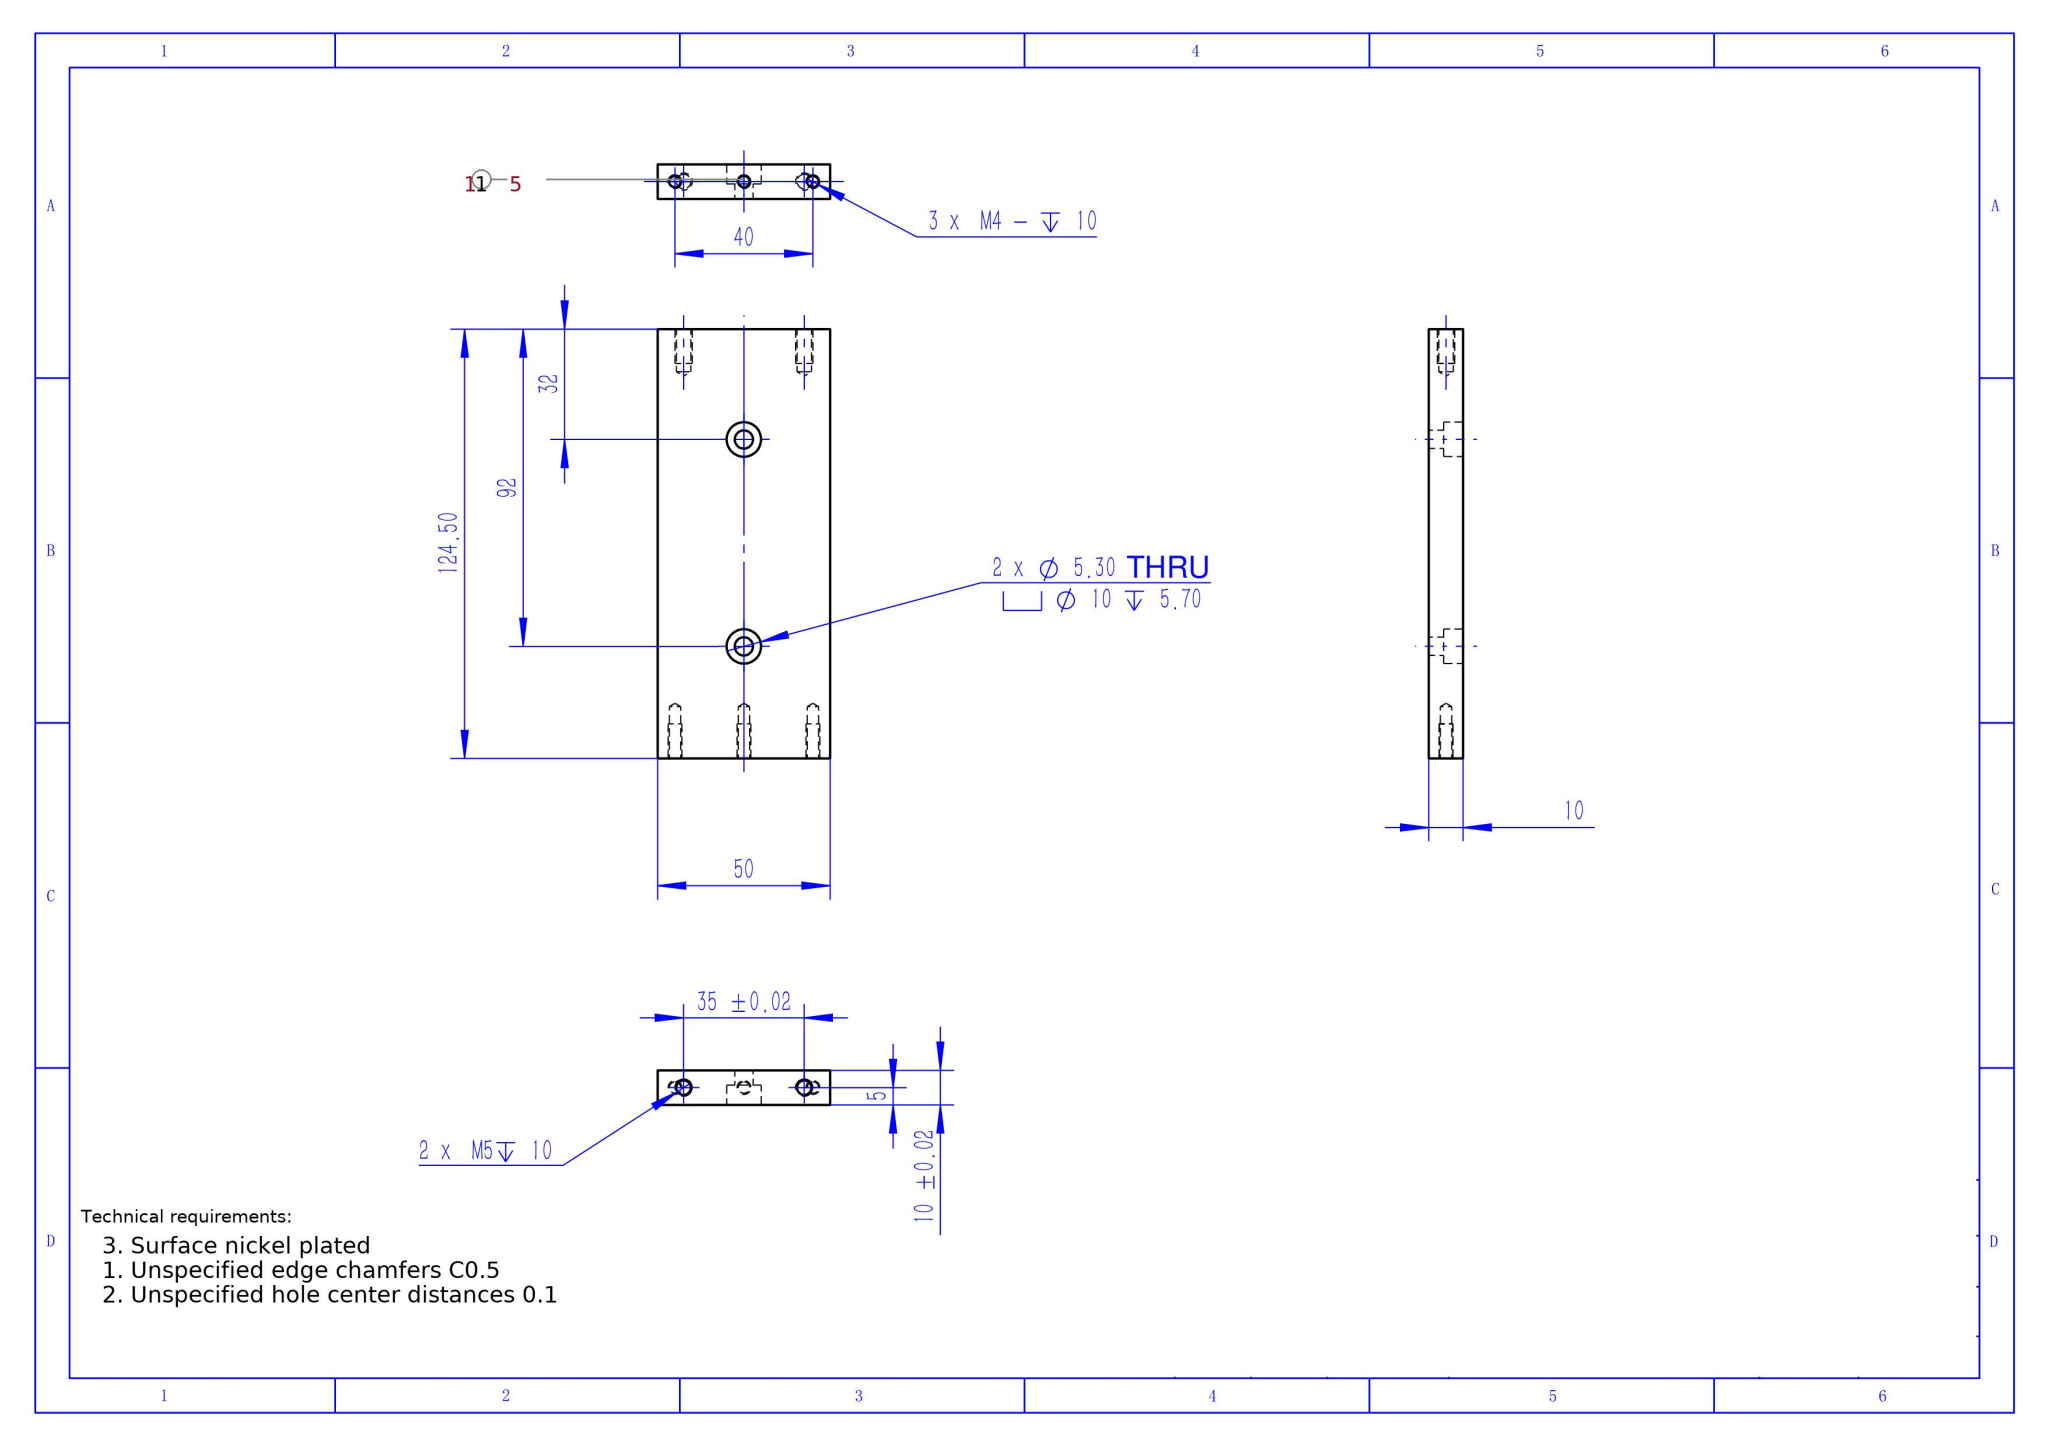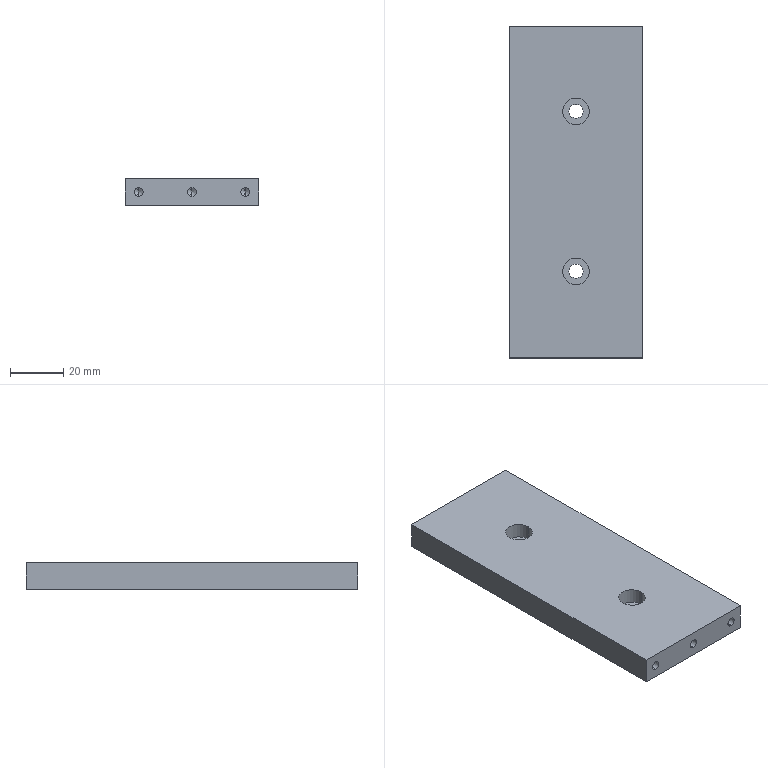Part | SolidWorks | mm | 1 solid | 36 faces | box 50 x 124.5 x 10 mm | volume 60416 mm3 | cylinder 18 | cone 10 | plane 8 | commonest cylinder face diameters 3.3 x6 10 x4 5.3 x4 4.2 x4
build123d program:
from build123d import *

# Parameters (mm, degrees)
SKETCH1_W                                         = 50
SKETCH1_H                                         = 124.5
BOSS_EXTRUDE1_DEPTH                               = 10
M5_TAPPED_HOLE1_D                                 = 4.2
M5_TAPPED_HOLE1_DEPTH                             = 12.4
M5_TAPPED_HOLE1_TIP                               = 1.262
HOLE_SIZE_ACCORDING_TO_HEX_SOCKET_HEA_D           = 5.3
HOLE_SIZE_ACCORDING_TO_HEX_SOCKET_HEA_CBORE_D     = 10
HOLE_SIZE_ACCORDING_TO_HEX_SOCKET_HEA_CBORE_DEPTH = 5.7
M4_TAPPED_HOLE1_D                                 = 3.3
M4_TAPPED_HOLE1_DEPTH                             = 15
M4_TAPPED_HOLE1_TIP                               = 0.9914


with BuildPart() as part:
    # Sketch1 → Boss-Extrude1 (new body)
    with BuildSketch(Plane.XY):
        with Locations((0, -62.25)):
            Rectangle(SKETCH1_W, SKETCH1_H)
    extrude(amount=BOSS_EXTRUDE1_DEPTH)

    # M5 Tapped Hole1
    with Locations(Plane(origin=(0, 0, 0), x_dir=(1, 0, 0), z_dir=(0, 1, 0))):
        with Locations((17.5, -5), (-17.5, -5)):
            Hole(M5_TAPPED_HOLE1_D / 2, depth=M5_TAPPED_HOLE1_DEPTH)
            with Locations((0, 0, -(M5_TAPPED_HOLE1_DEPTH + M5_TAPPED_HOLE1_TIP / 2))):  # 118° drill point
                Cone(0, M5_TAPPED_HOLE1_D / 2, M5_TAPPED_HOLE1_TIP, mode=Mode.SUBTRACT)

    # Hole Size _ according to_ Hex Socket Hea (through all)
    with Locations(Plane(origin=(0, 0, 10), x_dir=(-1, 0, 0), z_dir=(0, 0, 1))):
        with Locations((0, 32), (0, 92)):
            CounterBoreHole(HOLE_SIZE_ACCORDING_TO_HEX_SOCKET_HEA_D / 2, HOLE_SIZE_ACCORDING_TO_HEX_SOCKET_HEA_CBORE_D / 2, HOLE_SIZE_ACCORDING_TO_HEX_SOCKET_HEA_CBORE_DEPTH)

    # M4 Tapped Hole1
    with Locations(Plane(origin=(20, -124.5, 5), x_dir=(0, 0, -1), z_dir=(0, -1, 0))):
        with Locations((0, 0), (0, -20), (0, -40)):
            Hole(M4_TAPPED_HOLE1_D / 2, depth=M4_TAPPED_HOLE1_DEPTH)
            with Locations((0, 0, -(M4_TAPPED_HOLE1_DEPTH + M4_TAPPED_HOLE1_TIP / 2))):  # 118° drill point
                Cone(0, M4_TAPPED_HOLE1_D / 2, M4_TAPPED_HOLE1_TIP, mode=Mode.SUBTRACT)


solid = part.part
STEP:
#1=CARTESIAN_POINT('',(20.,-109.5,6.65));
#2=VERTEX_POINT('',#1);
#3=CARTESIAN_POINT('',(20.,-109.5,3.35));
#4=VERTEX_POINT('',#3);
#5=CARTESIAN_POINT('',(20.,-109.5,5.));
#6=DIRECTION('',(0.,-1.,0.));
#7=DIRECTION('',(0.,0.,-1.));
#8=AXIS2_PLACEMENT_3D('',#5,#6,#7);
#9=CIRCLE('',#8,1.65);
#10=EDGE_CURVE('',#2,#4,#9,.T.);
#11=ORIENTED_EDGE('',*,*,#10,.F.);
#12=CARTESIAN_POINT('',(20.,-124.5,6.65));
#13=VERTEX_POINT('',#12);
#14=CARTESIAN_POINT('',(20.,-124.5,6.65));
#15=DIRECTION('',(0.,-1.,0.));
#16=VECTOR('',#15,1000.);
#17=LINE('',#14,#16);
#18=EDGE_CURVE('',#2,#13,#17,.T.);
#19=ORIENTED_EDGE('',*,*,#18,.T.);
#20=CARTESIAN_POINT('',(20.,-124.5,3.35));
#21=VERTEX_POINT('',#20);
#22=CARTESIAN_POINT('',(20.,-124.5,5.));
#23=DIRECTION('',(0.,-1.,0.));
#24=DIRECTION('',(0.,0.,-1.));
#25=AXIS2_PLACEMENT_3D('',#22,#23,#24);
#26=CIRCLE('',#25,1.65);
#27=EDGE_CURVE('',#13,#21,#26,.T.);
#28=ORIENTED_EDGE('',*,*,#27,.T.);
#29=CARTESIAN_POINT('',(20.,-124.5,3.35));
#30=DIRECTION('',(0.,-1.,0.));
#31=VECTOR('',#30,1000.);
#32=LINE('',#29,#31);
#33=EDGE_CURVE('',#4,#21,#32,.T.);
#34=ORIENTED_EDGE('',*,*,#33,.F.);
#35=EDGE_LOOP('',(#11,#19,#28,#34));
#36=FACE_OUTER_BOUND('',#35,.T.);
#37=CARTESIAN_POINT('',(20.,-124.5,5.));
#38=DIRECTION('',(0.,-1.,0.));
#39=DIRECTION('',(0.,0.,-1.));
#40=AXIS2_PLACEMENT_3D('',#37,#38,#39);
#41=CYLINDRICAL_SURFACE('',#40,1.65);
#42=ADVANCED_FACE('',(#36),#41,.F.);
#43=CARTESIAN_POINT('',(20.,-108.509,5.));
#44=VERTEX_POINT('',#43);
#45=CARTESIAN_POINT('',(20.,-109.5,3.35));
#46=DIRECTION('',(0.,-0.515,-0.8572));
#47=VECTOR('',#46,1000.);
#48=LINE('',#45,#47);
#49=EDGE_CURVE('',#44,#4,#48,.T.);
#50=ORIENTED_EDGE('',*,*,#49,.F.);
#51=CARTESIAN_POINT('',(20.,-109.5,6.65));
#52=DIRECTION('',(0.,-0.515,0.8572));
#53=VECTOR('',#52,1000.);
#54=LINE('',#51,#53);
#55=EDGE_CURVE('',#44,#2,#54,.T.);
#56=ORIENTED_EDGE('',*,*,#55,.T.);
#57=ORIENTED_EDGE('',*,*,#10,.T.);
#58=EDGE_LOOP('',(#50,#56,#57));
#59=FACE_OUTER_BOUND('',#58,.T.);
#60=CARTESIAN_POINT('',(20.,-109.5,5.));
#61=DIRECTION('',(0.,-1.,0.));
#62=DIRECTION('',(0.,0.,-1.));
#63=AXIS2_PLACEMENT_3D('',#60,#61,#62);
#64=CONICAL_SURFACE('',#63,1.65,1.03);
#65=ADVANCED_FACE('',(#59),#64,.F.);
#66=CARTESIAN_POINT('',(-0.,-109.5,6.65));
#67=VERTEX_POINT('',#66);
#68=CARTESIAN_POINT('',(-0.,-109.5,3.35));
#69=VERTEX_POINT('',#68);
#70=CARTESIAN_POINT('',(-0.,-109.5,5.));
#71=DIRECTION('',(0.,-1.,0.));
#72=DIRECTION('',(0.,0.,-1.));
#73=AXIS2_PLACEMENT_3D('',#70,#71,#72);
#74=CIRCLE('',#73,1.65);
#75=EDGE_CURVE('',#67,#69,#74,.T.);
#76=ORIENTED_EDGE('',*,*,#75,.F.);
#77=CARTESIAN_POINT('',(-0.,-124.5,6.65));
#78=VERTEX_POINT('',#77);
#79=CARTESIAN_POINT('',(-0.,-124.5,6.65));
#80=DIRECTION('',(0.,-1.,0.));
#81=VECTOR('',#80,1000.);
#82=LINE('',#79,#81);
#83=EDGE_CURVE('',#67,#78,#82,.T.);
#84=ORIENTED_EDGE('',*,*,#83,.T.);
#85=CARTESIAN_POINT('',(-0.,-124.5,3.35));
#86=VERTEX_POINT('',#85);
#87=CARTESIAN_POINT('',(-0.,-124.5,5.));
#88=DIRECTION('',(0.,-1.,0.));
#89=DIRECTION('',(0.,0.,-1.));
#90=AXIS2_PLACEMENT_3D('',#87,#88,#89);
#91=CIRCLE('',#90,1.65);
#92=EDGE_CURVE('',#78,#86,#91,.T.);
#93=ORIENTED_EDGE('',*,*,#92,.T.);
#94=CARTESIAN_POINT('',(-0.,-124.5,3.35));
#95=DIRECTION('',(0.,-1.,0.));
#96=VECTOR('',#95,1000.);
#97=LINE('',#94,#96);
#98=EDGE_CURVE('',#69,#86,#97,.T.);
#99=ORIENTED_EDGE('',*,*,#98,.F.);
#100=EDGE_LOOP('',(#76,#84,#93,#99));
#101=FACE_OUTER_BOUND('',#100,.T.);
#102=CARTESIAN_POINT('',(-0.,-124.5,5.));
#103=DIRECTION('',(0.,-1.,0.));
#104=DIRECTION('',(0.,0.,-1.));
#105=AXIS2_PLACEMENT_3D('',#102,#103,#104);
#106=CYLINDRICAL_SURFACE('',#105,1.65);
#107=ADVANCED_FACE('',(#101),#106,.F.);
#108=CARTESIAN_POINT('',(-0.,-108.509,5.));
#109=VERTEX_POINT('',#108);
#110=CARTESIAN_POINT('',(-0.,-109.5,3.35));
#111=DIRECTION('',(0.,-0.515,-0.8572));
#112=VECTOR('',#111,1000.);
#113=LINE('',#110,#112);
#114=EDGE_CURVE('',#109,#69,#113,.T.);
#115=ORIENTED_EDGE('',*,*,#114,.F.);
#116=CARTESIAN_POINT('',(-0.,-109.5,6.65));
#117=DIRECTION('',(0.,-0.515,0.8572));
#118=VECTOR('',#117,1000.);
#119=LINE('',#116,#118);
#120=EDGE_CURVE('',#109,#67,#119,.T.);
#121=ORIENTED_EDGE('',*,*,#120,.T.);
#122=ORIENTED_EDGE('',*,*,#75,.T.);
#123=EDGE_LOOP('',(#115,#121,#122));
#124=FACE_OUTER_BOUND('',#123,.T.);
#125=CARTESIAN_POINT('',(-0.,-109.5,5.));
#126=DIRECTION('',(0.,-1.,0.));
#127=DIRECTION('',(0.,0.,-1.));
#128=AXIS2_PLACEMENT_3D('',#125,#126,#127);
#129=CONICAL_SURFACE('',#128,1.65,1.03);
#130=ADVANCED_FACE('',(#124),#129,.F.);
#131=CARTESIAN_POINT('',(-20.,-109.5,6.65));
#132=VERTEX_POINT('',#131);
#133=CARTESIAN_POINT('',(-20.,-109.5,3.35));
#134=VERTEX_POINT('',#133);
#135=CARTESIAN_POINT('',(-20.,-109.5,5.));
#136=DIRECTION('',(0.,-1.,0.));
#137=DIRECTION('',(0.,0.,-1.));
#138=AXIS2_PLACEMENT_3D('',#135,#136,#137);
#139=CIRCLE('',#138,1.65);
#140=EDGE_CURVE('',#132,#134,#139,.T.);
#141=ORIENTED_EDGE('',*,*,#140,.F.);
#142=CARTESIAN_POINT('',(-20.,-124.5,6.65));
#143=VERTEX_POINT('',#142);
#144=CARTESIAN_POINT('',(-20.,-124.5,6.65));
#145=DIRECTION('',(0.,-1.,0.));
#146=VECTOR('',#145,1000.);
#147=LINE('',#144,#146);
#148=EDGE_CURVE('',#132,#143,#147,.T.);
#149=ORIENTED_EDGE('',*,*,#148,.T.);
#150=CARTESIAN_POINT('',(-20.,-124.5,3.35));
#151=VERTEX_POINT('',#150);
#152=CARTESIAN_POINT('',(-20.,-124.5,5.));
#153=DIRECTION('',(0.,-1.,0.));
#154=DIRECTION('',(0.,0.,-1.));
#155=AXIS2_PLACEMENT_3D('',#152,#153,#154);
#156=CIRCLE('',#155,1.65);
#157=EDGE_CURVE('',#143,#151,#156,.T.);
#158=ORIENTED_EDGE('',*,*,#157,.T.);
#159=CARTESIAN_POINT('',(-20.,-124.5,3.35));
#160=DIRECTION('',(0.,-1.,0.));
#161=VECTOR('',#160,1000.);
#162=LINE('',#159,#161);
#163=EDGE_CURVE('',#134,#151,#162,.T.);
#164=ORIENTED_EDGE('',*,*,#163,.F.);
#165=EDGE_LOOP('',(#141,#149,#158,#164));
#166=FACE_OUTER_BOUND('',#165,.T.);
#167=CARTESIAN_POINT('',(-20.,-124.5,5.));
#168=DIRECTION('',(0.,-1.,0.));
#169=DIRECTION('',(0.,0.,-1.));
#170=AXIS2_PLACEMENT_3D('',#167,#168,#169);
#171=CYLINDRICAL_SURFACE('',#170,1.65);
#172=ADVANCED_FACE('',(#166),#171,.F.);
#173=CARTESIAN_POINT('',(-20.,-108.509,5.));
#174=VERTEX_POINT('',#173);
#175=CARTESIAN_POINT('',(-20.,-109.5,3.35));
#176=DIRECTION('',(0.,-0.515,-0.8572));
#177=VECTOR('',#176,1000.);
#178=LINE('',#175,#177);
#179=EDGE_CURVE('',#174,#134,#178,.T.);
#180=ORIENTED_EDGE('',*,*,#179,.F.);
#181=CARTESIAN_POINT('',(-20.,-109.5,6.65));
#182=DIRECTION('',(0.,-0.515,0.8572));
#183=VECTOR('',#182,1000.);
#184=LINE('',#181,#183);
#185=EDGE_CURVE('',#174,#132,#184,.T.);
#186=ORIENTED_EDGE('',*,*,#185,.T.);
#187=ORIENTED_EDGE('',*,*,#140,.T.);
#188=EDGE_LOOP('',(#180,#186,#187));
#189=FACE_OUTER_BOUND('',#188,.T.);
#190=CARTESIAN_POINT('',(-20.,-109.5,5.));
#191=DIRECTION('',(0.,-1.,0.));
#192=DIRECTION('',(0.,0.,-1.));
#193=AXIS2_PLACEMENT_3D('',#190,#191,#192);
#194=CONICAL_SURFACE('',#193,1.65,1.03);
#195=ADVANCED_FACE('',(#189),#194,.F.);
#196=CARTESIAN_POINT('',(-5.,-32.,4.3));
#197=VERTEX_POINT('',#196);
#198=CARTESIAN_POINT('',(5.,-32.,4.3));
#199=VERTEX_POINT('',#198);
#200=CARTESIAN_POINT('',(0.,-32.,4.3));
#201=DIRECTION('',(0.,0.,1.));
#202=DIRECTION('',(1.,0.,0.));
#203=AXIS2_PLACEMENT_3D('',#200,#201,#202);
#204=CIRCLE('',#203,5.);
#205=EDGE_CURVE('',#197,#199,#204,.T.);
#206=ORIENTED_EDGE('',*,*,#205,.F.);
#207=CARTESIAN_POINT('',(-5.,-32.,10.));
#208=VERTEX_POINT('',#207);
#209=CARTESIAN_POINT('',(-5.,-32.,10.));
#210=DIRECTION('',(0.,0.,1.));
#211=VECTOR('',#210,1000.);
#212=LINE('',#209,#211);
#213=EDGE_CURVE('',#197,#208,#212,.T.);
#214=ORIENTED_EDGE('',*,*,#213,.T.);
#215=CARTESIAN_POINT('',(5.,-32.,10.));
#216=VERTEX_POINT('',#215);
#217=CARTESIAN_POINT('',(0.,-32.,10.));
#218=DIRECTION('',(0.,0.,1.));
#219=DIRECTION('',(1.,0.,0.));
#220=AXIS2_PLACEMENT_3D('',#217,#218,#219);
#221=CIRCLE('',#220,5.);
#222=EDGE_CURVE('',#208,#216,#221,.T.);
#223=ORIENTED_EDGE('',*,*,#222,.T.);
#224=CARTESIAN_POINT('',(5.,-32.,10.));
#225=DIRECTION('',(0.,0.,1.));
#226=VECTOR('',#225,1000.);
#227=LINE('',#224,#226);
#228=EDGE_CURVE('',#199,#216,#227,.T.);
#229=ORIENTED_EDGE('',*,*,#228,.F.);
#230=EDGE_LOOP('',(#206,#214,#223,#229));
#231=FACE_OUTER_BOUND('',#230,.T.);
#232=CARTESIAN_POINT('',(0.,-32.,10.));
#233=DIRECTION('',(0.,0.,1.));
#234=DIRECTION('',(1.,0.,0.));
#235=AXIS2_PLACEMENT_3D('',#232,#233,#234);
#236=CYLINDRICAL_SURFACE('',#235,5.);
#237=ADVANCED_FACE('',(#231),#236,.F.);
#238=CARTESIAN_POINT('',(-2.65,-32.,0.));
#239=VERTEX_POINT('',#238);
#240=CARTESIAN_POINT('',(2.65,-32.,0.));
#241=VERTEX_POINT('',#240);
#242=CARTESIAN_POINT('',(0.,-32.,0.));
#243=DIRECTION('',(0.,0.,1.));
#244=DIRECTION('',(1.,0.,0.));
#245=AXIS2_PLACEMENT_3D('',#242,#243,#244);
#246=CIRCLE('',#245,2.65);
#247=EDGE_CURVE('',#239,#241,#246,.T.);
#248=ORIENTED_EDGE('',*,*,#247,.F.);
#249=CARTESIAN_POINT('',(-2.65,-32.,4.3));
#250=VERTEX_POINT('',#249);
#251=CARTESIAN_POINT('',(-2.65,-32.,10.));
#252=DIRECTION('',(0.,0.,1.));
#253=VECTOR('',#252,1000.);
#254=LINE('',#251,#253);
#255=EDGE_CURVE('',#239,#250,#254,.T.);
#256=ORIENTED_EDGE('',*,*,#255,.T.);
#257=CARTESIAN_POINT('',(2.65,-32.,4.3));
#258=VERTEX_POINT('',#257);
#259=CARTESIAN_POINT('',(0.,-32.,4.3));
#260=DIRECTION('',(0.,0.,1.));
#261=DIRECTION('',(1.,0.,0.));
#262=AXIS2_PLACEMENT_3D('',#259,#260,#261);
#263=CIRCLE('',#262,2.65);
#264=EDGE_CURVE('',#250,#258,#263,.T.);
#265=ORIENTED_EDGE('',*,*,#264,.T.);
#266=CARTESIAN_POINT('',(2.65,-32.,10.));
#267=DIRECTION('',(0.,0.,1.));
#268=VECTOR('',#267,1000.);
#269=LINE('',#266,#268);
#270=EDGE_CURVE('',#241,#258,#269,.T.);
#271=ORIENTED_EDGE('',*,*,#270,.F.);
#272=EDGE_LOOP('',(#248,#256,#265,#271));
#273=FACE_OUTER_BOUND('',#272,.T.);
#274=CARTESIAN_POINT('',(0.,-32.,10.));
#275=DIRECTION('',(0.,0.,1.));
#276=DIRECTION('',(1.,0.,0.));
#277=AXIS2_PLACEMENT_3D('',#274,#275,#276);
#278=CYLINDRICAL_SURFACE('',#277,2.65);
#279=ADVANCED_FACE('',(#273),#278,.F.);
#280=CARTESIAN_POINT('',(-5.,-92.,4.3));
#281=VERTEX_POINT('',#280);
#282=CARTESIAN_POINT('',(5.,-92.,4.3));
#283=VERTEX_POINT('',#282);
#284=CARTESIAN_POINT('',(0.,-92.,4.3));
#285=DIRECTION('',(0.,0.,1.));
#286=DIRECTION('',(1.,0.,0.));
#287=AXIS2_PLACEMENT_3D('',#284,#285,#286);
#288=CIRCLE('',#287,5.);
#289=EDGE_CURVE('',#281,#283,#288,.T.);
#290=ORIENTED_EDGE('',*,*,#289,.F.);
#291=CARTESIAN_POINT('',(-5.,-92.,10.));
#292=VERTEX_POINT('',#291);
#293=CARTESIAN_POINT('',(-5.,-92.,10.));
#294=DIRECTION('',(0.,0.,1.));
#295=VECTOR('',#294,1000.);
#296=LINE('',#293,#295);
#297=EDGE_CURVE('',#281,#292,#296,.T.);
#298=ORIENTED_EDGE('',*,*,#297,.T.);
#299=CARTESIAN_POINT('',(5.,-92.,10.));
#300=VERTEX_POINT('',#299);
#301=CARTESIAN_POINT('',(0.,-92.,10.));
#302=DIRECTION('',(0.,0.,1.));
#303=DIRECTION('',(1.,0.,0.));
#304=AXIS2_PLACEMENT_3D('',#301,#302,#303);
#305=CIRCLE('',#304,5.);
#306=EDGE_CURVE('',#292,#300,#305,.T.);
#307=ORIENTED_EDGE('',*,*,#306,.T.);
#308=CARTESIAN_POINT('',(5.,-92.,10.));
#309=DIRECTION('',(0.,0.,1.));
#310=VECTOR('',#309,1000.);
#311=LINE('',#308,#310);
#312=EDGE_CURVE('',#283,#300,#311,.T.);
#313=ORIENTED_EDGE('',*,*,#312,.F.);
#314=EDGE_LOOP('',(#290,#298,#307,#313));
#315=FACE_OUTER_BOUND('',#314,.T.);
#316=CARTESIAN_POINT('',(0.,-92.,10.));
#317=DIRECTION('',(0.,0.,1.));
#318=DIRECTION('',(1.,0.,0.));
#319=AXIS2_PLACEMENT_3D('',#316,#317,#318);
#320=CYLINDRICAL_SURFACE('',#319,5.);
#321=ADVANCED_FACE('',(#315),#320,.F.);
#322=CARTESIAN_POINT('',(-2.65,-92.,0.));
#323=VERTEX_POINT('',#322);
#324=CARTESIAN_POINT('',(2.65,-92.,0.));
#325=VERTEX_POINT('',#324);
#326=CARTESIAN_POINT('',(0.,-92.,0.));
#327=DIRECTION('',(0.,0.,1.));
#328=DIRECTION('',(1.,0.,0.));
#329=AXIS2_PLACEMENT_3D('',#326,#327,#328);
#330=CIRCLE('',#329,2.65);
#331=EDGE_CURVE('',#323,#325,#330,.T.);
#332=ORIENTED_EDGE('',*,*,#331,.F.);
#333=CARTESIAN_POINT('',(-2.65,-92.,4.3));
#334=VERTEX_POINT('',#333);
#335=CARTESIAN_POINT('',(-2.65,-92.,10.));
#336=DIRECTION('',(0.,0.,1.));
#337=VECTOR('',#336,1000.);
#338=LINE('',#335,#337);
#339=EDGE_CURVE('',#323,#334,#338,.T.);
#340=ORIENTED_EDGE('',*,*,#339,.T.);
#341=CARTESIAN_POINT('',(2.65,-92.,4.3));
#342=VERTEX_POINT('',#341);
#343=CARTESIAN_POINT('',(0.,-92.,4.3));
#344=DIRECTION('',(0.,0.,1.));
#345=DIRECTION('',(1.,0.,0.));
#346=AXIS2_PLACEMENT_3D('',#343,#344,#345);
#347=CIRCLE('',#346,2.65);
#348=EDGE_CURVE('',#334,#342,#347,.T.);
#349=ORIENTED_EDGE('',*,*,#348,.T.);
#350=CARTESIAN_POINT('',(2.65,-92.,10.));
#351=DIRECTION('',(0.,0.,1.));
#352=VECTOR('',#351,1000.);
#353=LINE('',#350,#352);
#354=EDGE_CURVE('',#325,#342,#353,.T.);
#355=ORIENTED_EDGE('',*,*,#354,.F.);
#356=EDGE_LOOP('',(#332,#340,#349,#355));
#357=FACE_OUTER_BOUND('',#356,.T.);
#358=CARTESIAN_POINT('',(0.,-92.,10.));
#359=DIRECTION('',(0.,0.,1.));
#360=DIRECTION('',(1.,0.,0.));
#361=AXIS2_PLACEMENT_3D('',#358,#359,#360);
#362=CYLINDRICAL_SURFACE('',#361,2.65);
#363=ADVANCED_FACE('',(#357),#362,.F.);
#364=CARTESIAN_POINT('',(17.5,-12.4,2.9));
#365=VERTEX_POINT('',#364);
#366=CARTESIAN_POINT('',(17.5,-12.4,7.1));
#367=VERTEX_POINT('',#366);
#368=CARTESIAN_POINT('',(17.5,-12.4,5.));
#369=DIRECTION('',(0.,1.,0.));
#370=DIRECTION('',(0.,0.,1.));
#371=AXIS2_PLACEMENT_3D('',#368,#369,#370);
#372=CIRCLE('',#371,2.1);
#373=EDGE_CURVE('',#365,#367,#372,.T.);
#374=ORIENTED_EDGE('',*,*,#373,.F.);
#375=CARTESIAN_POINT('',(17.5,0.,2.9));
#376=VERTEX_POINT('',#375);
#377=CARTESIAN_POINT('',(17.5,0.,2.9));
#378=DIRECTION('',(0.,1.,0.));
#379=VECTOR('',#378,1000.);
#380=LINE('',#377,#379);
#381=EDGE_CURVE('',#365,#376,#380,.T.);
#382=ORIENTED_EDGE('',*,*,#381,.T.);
#383=CARTESIAN_POINT('',(17.5,0.,7.1));
#384=VERTEX_POINT('',#383);
#385=CARTESIAN_POINT('',(17.5,0.,5.));
#386=DIRECTION('',(0.,1.,0.));
#387=DIRECTION('',(0.,0.,1.));
#388=AXIS2_PLACEMENT_3D('',#385,#386,#387);
#389=CIRCLE('',#388,2.1);
#390=EDGE_CURVE('',#376,#384,#389,.T.);
#391=ORIENTED_EDGE('',*,*,#390,.T.);
#392=CARTESIAN_POINT('',(17.5,0.,7.1));
#393=DIRECTION('',(0.,1.,0.));
#394=VECTOR('',#393,1000.);
#395=LINE('',#392,#394);
#396=EDGE_CURVE('',#367,#384,#395,.T.);
#397=ORIENTED_EDGE('',*,*,#396,.F.);
#398=EDGE_LOOP('',(#374,#382,#391,#397));
#399=FACE_OUTER_BOUND('',#398,.T.);
#400=CARTESIAN_POINT('',(17.5,0.,5.));
#401=DIRECTION('',(0.,1.,0.));
#402=DIRECTION('',(0.,0.,1.));
#403=AXIS2_PLACEMENT_3D('',#400,#401,#402);
#404=CYLINDRICAL_SURFACE('',#403,2.1);
#405=ADVANCED_FACE('',(#399),#404,.F.);
#406=CARTESIAN_POINT('',(17.5,-13.662,5.));
#407=VERTEX_POINT('',#406);
#408=CARTESIAN_POINT('',(17.5,-12.4,7.1));
#409=DIRECTION('',(0.,0.515,0.8572));
#410=VECTOR('',#409,1000.);
#411=LINE('',#408,#410);
#412=EDGE_CURVE('',#407,#367,#411,.T.);
#413=ORIENTED_EDGE('',*,*,#412,.F.);
#414=CARTESIAN_POINT('',(17.5,-12.4,2.9));
#415=DIRECTION('',(0.,0.515,-0.8572));
#416=VECTOR('',#415,1000.);
#417=LINE('',#414,#416);
#418=EDGE_CURVE('',#407,#365,#417,.T.);
#419=ORIENTED_EDGE('',*,*,#418,.T.);
#420=ORIENTED_EDGE('',*,*,#373,.T.);
#421=EDGE_LOOP('',(#413,#419,#420));
#422=FACE_OUTER_BOUND('',#421,.T.);
#423=CARTESIAN_POINT('',(17.5,-12.4,5.));
#424=DIRECTION('',(0.,1.,0.));
#425=DIRECTION('',(0.,0.,1.));
#426=AXIS2_PLACEMENT_3D('',#423,#424,#425);
#427=CONICAL_SURFACE('',#426,2.1,1.03);
#428=ADVANCED_FACE('',(#422),#427,.F.);
#429=CARTESIAN_POINT('',(-17.5,-12.4,2.9));
#430=VERTEX_POINT('',#429);
#431=CARTESIAN_POINT('',(-17.5,-12.4,7.1));
#432=VERTEX_POINT('',#431);
#433=CARTESIAN_POINT('',(-17.5,-12.4,5.));
#434=DIRECTION('',(0.,1.,0.));
#435=DIRECTION('',(0.,0.,1.));
#436=AXIS2_PLACEMENT_3D('',#433,#434,#435);
#437=CIRCLE('',#436,2.1);
#438=EDGE_CURVE('',#430,#432,#437,.T.);
#439=ORIENTED_EDGE('',*,*,#438,.F.);
#440=CARTESIAN_POINT('',(-17.5,0.,2.9));
#441=VERTEX_POINT('',#440);
#442=CARTESIAN_POINT('',(-17.5,0.,2.9));
#443=DIRECTION('',(0.,1.,0.));
#444=VECTOR('',#443,1000.);
#445=LINE('',#442,#444);
#446=EDGE_CURVE('',#430,#441,#445,.T.);
#447=ORIENTED_EDGE('',*,*,#446,.T.);
#448=CARTESIAN_POINT('',(-17.5,0.,7.1));
#449=VERTEX_POINT('',#448);
#450=CARTESIAN_POINT('',(-17.5,0.,5.));
#451=DIRECTION('',(0.,1.,0.));
#452=DIRECTION('',(0.,0.,1.));
#453=AXIS2_PLACEMENT_3D('',#450,#451,#452);
#454=CIRCLE('',#453,2.1);
#455=EDGE_CURVE('',#441,#449,#454,.T.);
#456=ORIENTED_EDGE('',*,*,#455,.T.);
#457=CARTESIAN_POINT('',(-17.5,0.,7.1));
#458=DIRECTION('',(0.,1.,0.));
#459=VECTOR('',#458,1000.);
#460=LINE('',#457,#459);
#461=EDGE_CURVE('',#432,#449,#460,.T.);
#462=ORIENTED_EDGE('',*,*,#461,.F.);
#463=EDGE_LOOP('',(#439,#447,#456,#462));
#464=FACE_OUTER_BOUND('',#463,.T.);
#465=CARTESIAN_POINT('',(-17.5,0.,5.));
#466=DIRECTION('',(0.,1.,0.));
#467=DIRECTION('',(0.,0.,1.));
#468=AXIS2_PLACEMENT_3D('',#465,#466,#467);
#469=CYLINDRICAL_SURFACE('',#468,2.1);
#470=ADVANCED_FACE('',(#464),#469,.F.);
#471=CARTESIAN_POINT('',(-17.5,-13.662,5.));
#472=VERTEX_POINT('',#471);
#473=CARTESIAN_POINT('',(-17.5,-12.4,7.1));
#474=DIRECTION('',(0.,0.515,0.8572));
#475=VECTOR('',#474,1000.);
#476=LINE('',#473,#475);
#477=EDGE_CURVE('',#472,#432,#476,.T.);
#478=ORIENTED_EDGE('',*,*,#477,.F.);
#479=CARTESIAN_POINT('',(-17.5,-12.4,2.9));
#480=DIRECTION('',(0.,0.515,-0.8572));
#481=VECTOR('',#480,1000.);
#482=LINE('',#479,#481);
#483=EDGE_CURVE('',#472,#430,#482,.T.);
#484=ORIENTED_EDGE('',*,*,#483,.T.);
#485=ORIENTED_EDGE('',*,*,#438,.T.);
#486=EDGE_LOOP('',(#478,#484,#485));
#487=FACE_OUTER_BOUND('',#486,.T.);
#488=CARTESIAN_POINT('',(-17.5,-12.4,5.));
#489=DIRECTION('',(0.,1.,0.));
#490=DIRECTION('',(0.,0.,1.));
#491=AXIS2_PLACEMENT_3D('',#488,#489,#490);
#492=CONICAL_SURFACE('',#491,2.1,1.03);
#493=ADVANCED_FACE('',(#487),#492,.F.);
#494=CARTESIAN_POINT('',(-25.,0.,0.));
#495=VERTEX_POINT('',#494);
#496=CARTESIAN_POINT('',(-25.,-124.5,0.));
#497=VERTEX_POINT('',#496);
#498=CARTESIAN_POINT('',(-25.,0.,0.));
#499=DIRECTION('',(-0.,-1.,0.));
#500=VECTOR('',#499,1000.);
#501=LINE('',#498,#500);
#502=EDGE_CURVE('',#495,#497,#501,.T.);
#503=ORIENTED_EDGE('',*,*,#502,.T.);
#504=CARTESIAN_POINT('',(-25.,-124.5,10.));
#505=VERTEX_POINT('',#504);
#506=CARTESIAN_POINT('',(-25.,-124.5,10.));
#507=DIRECTION('',(0.,0.,-1.));
#508=VECTOR('',#507,1000.);
#509=LINE('',#506,#508);
#510=EDGE_CURVE('',#505,#497,#509,.T.);
#511=ORIENTED_EDGE('',*,*,#510,.F.);
#512=CARTESIAN_POINT('',(-25.,0.,10.));
#513=VERTEX_POINT('',#512);
#514=CARTESIAN_POINT('',(-25.,0.,10.));
#515=DIRECTION('',(-0.,-1.,0.));
#516=VECTOR('',#515,1000.);
#517=LINE('',#514,#516);
#518=EDGE_CURVE('',#513,#505,#517,.T.);
#519=ORIENTED_EDGE('',*,*,#518,.F.);
#520=CARTESIAN_POINT('',(-25.,0.,10.));
#521=DIRECTION('',(0.,0.,-1.));
#522=VECTOR('',#521,1000.);
#523=LINE('',#520,#522);
#524=EDGE_CURVE('',#513,#495,#523,.T.);
#525=ORIENTED_EDGE('',*,*,#524,.T.);
#526=EDGE_LOOP('',(#503,#511,#519,#525));
#527=FACE_OUTER_BOUND('',#526,.T.);
#528=CARTESIAN_POINT('',(-25.,0.,10.));
#529=DIRECTION('',(1.,-0.,0.));
#530=DIRECTION('',(0.,1.,0.));
#531=AXIS2_PLACEMENT_3D('',#528,#529,#530);
#532=PLANE('',#531);
#533=ADVANCED_FACE('',(#527),#532,.F.);
#534=CARTESIAN_POINT('',(20.,-124.5,5.));
#535=DIRECTION('',(0.,-1.,0.));
#536=DIRECTION('',(0.,0.,-1.));
#537=AXIS2_PLACEMENT_3D('',#534,#535,#536);
#538=CIRCLE('',#537,1.65);
#539=EDGE_CURVE('',#21,#13,#538,.T.);
#540=ORIENTED_EDGE('',*,*,#539,.F.);
#541=ORIENTED_EDGE('',*,*,#27,.F.);
#542=EDGE_LOOP('',(#540,#541));
#543=FACE_BOUND('',#542,.T.);
#544=CARTESIAN_POINT('',(-0.,-124.5,5.));
#545=DIRECTION('',(0.,-1.,0.));
#546=DIRECTION('',(0.,0.,-1.));
#547=AXIS2_PLACEMENT_3D('',#544,#545,#546);
#548=CIRCLE('',#547,1.65);
#549=EDGE_CURVE('',#86,#78,#548,.T.);
#550=ORIENTED_EDGE('',*,*,#549,.F.);
#551=ORIENTED_EDGE('',*,*,#92,.F.);
#552=EDGE_LOOP('',(#550,#551));
#553=FACE_BOUND('',#552,.T.);
#554=CARTESIAN_POINT('',(-20.,-124.5,5.));
#555=DIRECTION('',(0.,-1.,0.));
#556=DIRECTION('',(0.,0.,-1.));
#557=AXIS2_PLACEMENT_3D('',#554,#555,#556);
#558=CIRCLE('',#557,1.65);
#559=EDGE_CURVE('',#151,#143,#558,.T.);
#560=ORIENTED_EDGE('',*,*,#559,.F.);
#561=ORIENTED_EDGE('',*,*,#157,.F.);
#562=EDGE_LOOP('',(#560,#561));
#563=FACE_BOUND('',#562,.T.);
#564=CARTESIAN_POINT('',(25.,-124.5,0.));
#565=VERTEX_POINT('',#564);
#566=CARTESIAN_POINT('',(-25.,-124.5,0.));
#567=DIRECTION('',(1.,0.,0.));
#568=VECTOR('',#567,1000.);
#569=LINE('',#566,#568);
#570=EDGE_CURVE('',#497,#565,#569,.T.);
#571=ORIENTED_EDGE('',*,*,#570,.T.);
#572=CARTESIAN_POINT('',(25.,-124.5,10.));
#573=VERTEX_POINT('',#572);
#574=CARTESIAN_POINT('',(25.,-124.5,10.));
#575=DIRECTION('',(0.,0.,-1.));
#576=VECTOR('',#575,1000.);
#577=LINE('',#574,#576);
#578=EDGE_CURVE('',#573,#565,#577,.T.);
#579=ORIENTED_EDGE('',*,*,#578,.F.);
#580=CARTESIAN_POINT('',(-25.,-124.5,10.));
#581=DIRECTION('',(1.,0.,0.));
#582=VECTOR('',#581,1000.);
#583=LINE('',#580,#582);
#584=EDGE_CURVE('',#505,#573,#583,.T.);
#585=ORIENTED_EDGE('',*,*,#584,.F.);
#586=ORIENTED_EDGE('',*,*,#510,.T.);
#587=EDGE_LOOP('',(#571,#579,#585,#586));
#588=FACE_OUTER_BOUND('',#587,.T.);
#589=CARTESIAN_POINT('',(-25.,-124.5,10.));
#590=DIRECTION('',(0.,1.,0.));
#591=DIRECTION('',(0.,0.,1.));
#592=AXIS2_PLACEMENT_3D('',#589,#590,#591);
#593=PLANE('',#592);
#594=ADVANCED_FACE('',(#543,#553,#563,#588),#593,.F.);
#595=CARTESIAN_POINT('',(25.,0.,0.));
#596=VERTEX_POINT('',#595);
#597=CARTESIAN_POINT('',(25.,0.,0.));
#598=DIRECTION('',(-0.,1.,0.));
#599=VECTOR('',#598,1000.);
#600=LINE('',#597,#599);
#601=EDGE_CURVE('',#565,#596,#600,.T.);
#602=ORIENTED_EDGE('',*,*,#601,.T.);
#603=CARTESIAN_POINT('',(25.,0.,10.));
#604=VERTEX_POINT('',#603);
#605=CARTESIAN_POINT('',(25.,0.,10.));
#606=DIRECTION('',(0.,0.,-1.));
#607=VECTOR('',#606,1000.);
#608=LINE('',#605,#607);
#609=EDGE_CURVE('',#604,#596,#608,.T.);
#610=ORIENTED_EDGE('',*,*,#609,.F.);
#611=CARTESIAN_POINT('',(25.,0.,10.));
#612=DIRECTION('',(-0.,1.,0.));
#613=VECTOR('',#612,1000.);
#614=LINE('',#611,#613);
#615=EDGE_CURVE('',#573,#604,#614,.T.);
#616=ORIENTED_EDGE('',*,*,#615,.F.);
#617=ORIENTED_EDGE('',*,*,#578,.T.);
#618=EDGE_LOOP('',(#602,#610,#616,#617));
#619=FACE_OUTER_BOUND('',#618,.T.);
#620=CARTESIAN_POINT('',(25.,0.,10.));
#621=DIRECTION('',(-1.,-0.,0.));
#622=DIRECTION('',(0.,-1.,0.));
#623=AXIS2_PLACEMENT_3D('',#620,#621,#622);
#624=PLANE('',#623);
#625=ADVANCED_FACE('',(#619),#624,.F.);
#626=CARTESIAN_POINT('',(17.5,0.,5.));
#627=DIRECTION('',(0.,1.,0.));
#628=DIRECTION('',(0.,0.,1.));
#629=AXIS2_PLACEMENT_3D('',#626,#627,#628);
#630=CIRCLE('',#629,2.1);
#631=EDGE_CURVE('',#384,#376,#630,.T.);
#632=ORIENTED_EDGE('',*,*,#631,.F.);
#633=ORIENTED_EDGE('',*,*,#390,.F.);
#634=EDGE_LOOP('',(#632,#633));
#635=FACE_BOUND('',#634,.T.);
#636=CARTESIAN_POINT('',(-17.5,0.,5.));
#637=DIRECTION('',(0.,1.,0.));
#638=DIRECTION('',(0.,0.,1.));
#639=AXIS2_PLACEMENT_3D('',#636,#637,#638);
#640=CIRCLE('',#639,2.1);
#641=EDGE_CURVE('',#449,#441,#640,.T.);
#642=ORIENTED_EDGE('',*,*,#641,.F.);
#643=ORIENTED_EDGE('',*,*,#455,.F.);
#644=EDGE_LOOP('',(#642,#643));
#645=FACE_BOUND('',#644,.T.);
#646=CARTESIAN_POINT('',(-25.,0.,0.));
#647=DIRECTION('',(-1.,0.,0.));
#648=VECTOR('',#647,1000.);
#649=LINE('',#646,#648);
#650=EDGE_CURVE('',#596,#495,#649,.T.);
#651=ORIENTED_EDGE('',*,*,#650,.T.);
#652=ORIENTED_EDGE('',*,*,#524,.F.);
#653=CARTESIAN_POINT('',(-25.,0.,10.));
#654=DIRECTION('',(-1.,0.,0.));
#655=VECTOR('',#654,1000.);
#656=LINE('',#653,#655);
#657=EDGE_CURVE('',#604,#513,#656,.T.);
#658=ORIENTED_EDGE('',*,*,#657,.F.);
#659=ORIENTED_EDGE('',*,*,#609,.T.);
#660=EDGE_LOOP('',(#651,#652,#658,#659));
#661=FACE_OUTER_BOUND('',#660,.T.);
#662=CARTESIAN_POINT('',(-25.,0.,10.));
#663=DIRECTION('',(0.,-1.,0.));
#664=DIRECTION('',(0.,0.,-1.));
#665=AXIS2_PLACEMENT_3D('',#662,#663,#664);
#666=PLANE('',#665);
#667=ADVANCED_FACE('',(#635,#645,#661),#666,.F.);
#668=CARTESIAN_POINT('',(0.,-32.,10.));
#669=DIRECTION('',(0.,0.,1.));
#670=DIRECTION('',(1.,0.,0.));
#671=AXIS2_PLACEMENT_3D('',#668,#669,#670);
#672=CIRCLE('',#671,5.);
#673=EDGE_CURVE('',#216,#208,#672,.T.);
#674=ORIENTED_EDGE('',*,*,#673,.F.);
#675=ORIENTED_EDGE('',*,*,#222,.F.);
#676=EDGE_LOOP('',(#674,#675));
#677=FACE_BOUND('',#676,.T.);
#678=CARTESIAN_POINT('',(0.,-92.,10.));
#679=DIRECTION('',(0.,0.,1.));
#680=DIRECTION('',(1.,0.,0.));
#681=AXIS2_PLACEMENT_3D('',#678,#679,#680);
#682=CIRCLE('',#681,5.);
#683=EDGE_CURVE('',#300,#292,#682,.T.);
#684=ORIENTED_EDGE('',*,*,#683,.F.);
#685=ORIENTED_EDGE('',*,*,#306,.F.);
#686=EDGE_LOOP('',(#684,#685));
#687=FACE_BOUND('',#686,.T.);
#688=ORIENTED_EDGE('',*,*,#518,.T.);
#689=ORIENTED_EDGE('',*,*,#584,.T.);
#690=ORIENTED_EDGE('',*,*,#615,.T.);
#691=ORIENTED_EDGE('',*,*,#657,.T.);
#692=EDGE_LOOP('',(#688,#689,#690,#691));
#693=FACE_OUTER_BOUND('',#692,.T.);
#694=CARTESIAN_POINT('',(0.,0.,10.));
#695=DIRECTION('',(0.,0.,1.));
#696=DIRECTION('',(1.,0.,0.));
#697=AXIS2_PLACEMENT_3D('',#694,#695,#696);
#698=PLANE('',#697);
#699=ADVANCED_FACE('',(#677,#687,#693),#698,.T.);
#700=CARTESIAN_POINT('',(0.,-32.,0.));
#701=DIRECTION('',(0.,0.,1.));
#702=DIRECTION('',(1.,0.,0.));
#703=AXIS2_PLACEMENT_3D('',#700,#701,#702);
#704=CIRCLE('',#703,2.65);
#705=EDGE_CURVE('',#241,#239,#704,.T.);
#706=ORIENTED_EDGE('',*,*,#705,.T.);
#707=ORIENTED_EDGE('',*,*,#247,.T.);
#708=EDGE_LOOP('',(#706,#707));
#709=FACE_BOUND('',#708,.T.);
#710=CARTESIAN_POINT('',(0.,-92.,0.));
#711=DIRECTION('',(0.,0.,1.));
#712=DIRECTION('',(1.,0.,0.));
#713=AXIS2_PLACEMENT_3D('',#710,#711,#712);
#714=CIRCLE('',#713,2.65);
#715=EDGE_CURVE('',#325,#323,#714,.T.);
#716=ORIENTED_EDGE('',*,*,#715,.T.);
#717=ORIENTED_EDGE('',*,*,#331,.T.);
#718=EDGE_LOOP('',(#716,#717));
#719=FACE_BOUND('',#718,.T.);
#720=ORIENTED_EDGE('',*,*,#502,.F.);
#721=ORIENTED_EDGE('',*,*,#650,.F.);
#722=ORIENTED_EDGE('',*,*,#601,.F.);
#723=ORIENTED_EDGE('',*,*,#570,.F.);
#724=EDGE_LOOP('',(#720,#721,#722,#723));
#725=FACE_OUTER_BOUND('',#724,.T.);
#726=CARTESIAN_POINT('',(0.,0.,0.));
#727=DIRECTION('',(0.,0.,1.));
#728=DIRECTION('',(1.,0.,0.));
#729=AXIS2_PLACEMENT_3D('',#726,#727,#728);
#730=PLANE('',#729);
#731=ADVANCED_FACE('',(#709,#719,#725),#730,.F.);
#732=ORIENTED_EDGE('',*,*,#483,.F.);
#733=ORIENTED_EDGE('',*,*,#477,.T.);
#734=CARTESIAN_POINT('',(-17.5,-12.4,5.));
#735=DIRECTION('',(0.,1.,0.));
#736=DIRECTION('',(0.,0.,1.));
#737=AXIS2_PLACEMENT_3D('',#734,#735,#736);
#738=CIRCLE('',#737,2.1);
#739=EDGE_CURVE('',#432,#430,#738,.T.);
#740=ORIENTED_EDGE('',*,*,#739,.T.);
#741=EDGE_LOOP('',(#732,#733,#740));
#742=FACE_OUTER_BOUND('',#741,.T.);
#743=CARTESIAN_POINT('',(-17.5,-12.4,5.));
#744=DIRECTION('',(0.,1.,0.));
#745=DIRECTION('',(0.,0.,1.));
#746=AXIS2_PLACEMENT_3D('',#743,#744,#745);
#747=CONICAL_SURFACE('',#746,2.1,1.03);
#748=ADVANCED_FACE('',(#742),#747,.F.);
#749=ORIENTED_EDGE('',*,*,#446,.F.);
#750=ORIENTED_EDGE('',*,*,#739,.F.);
#751=ORIENTED_EDGE('',*,*,#461,.T.);
#752=ORIENTED_EDGE('',*,*,#641,.T.);
#753=EDGE_LOOP('',(#749,#750,#751,#752));
#754=FACE_OUTER_BOUND('',#753,.T.);
#755=CARTESIAN_POINT('',(-17.5,0.,5.));
#756=DIRECTION('',(0.,1.,0.));
#757=DIRECTION('',(0.,0.,1.));
#758=AXIS2_PLACEMENT_3D('',#755,#756,#757);
#759=CYLINDRICAL_SURFACE('',#758,2.1);
#760=ADVANCED_FACE('',(#754),#759,.F.);
#761=ORIENTED_EDGE('',*,*,#418,.F.);
#762=ORIENTED_EDGE('',*,*,#412,.T.);
#763=CARTESIAN_POINT('',(17.5,-12.4,5.));
#764=DIRECTION('',(0.,1.,0.));
#765=DIRECTION('',(0.,0.,1.));
#766=AXIS2_PLACEMENT_3D('',#763,#764,#765);
#767=CIRCLE('',#766,2.1);
#768=EDGE_CURVE('',#367,#365,#767,.T.);
#769=ORIENTED_EDGE('',*,*,#768,.T.);
#770=EDGE_LOOP('',(#761,#762,#769));
#771=FACE_OUTER_BOUND('',#770,.T.);
#772=CARTESIAN_POINT('',(17.5,-12.4,5.));
#773=DIRECTION('',(0.,1.,0.));
#774=DIRECTION('',(0.,0.,1.));
#775=AXIS2_PLACEMENT_3D('',#772,#773,#774);
#776=CONICAL_SURFACE('',#775,2.1,1.03);
#777=ADVANCED_FACE('',(#771),#776,.F.);
#778=ORIENTED_EDGE('',*,*,#381,.F.);
#779=ORIENTED_EDGE('',*,*,#768,.F.);
#780=ORIENTED_EDGE('',*,*,#396,.T.);
#781=ORIENTED_EDGE('',*,*,#631,.T.);
#782=EDGE_LOOP('',(#778,#779,#780,#781));
#783=FACE_OUTER_BOUND('',#782,.T.);
#784=CARTESIAN_POINT('',(17.5,0.,5.));
#785=DIRECTION('',(0.,1.,0.));
#786=DIRECTION('',(0.,0.,1.));
#787=AXIS2_PLACEMENT_3D('',#784,#785,#786);
#788=CYLINDRICAL_SURFACE('',#787,2.1);
#789=ADVANCED_FACE('',(#783),#788,.F.);
#790=ORIENTED_EDGE('',*,*,#339,.F.);
#791=ORIENTED_EDGE('',*,*,#715,.F.);
#792=ORIENTED_EDGE('',*,*,#354,.T.);
#793=CARTESIAN_POINT('',(0.,-92.,4.3));
#794=DIRECTION('',(0.,0.,1.));
#795=DIRECTION('',(1.,0.,0.));
#796=AXIS2_PLACEMENT_3D('',#793,#794,#795);
#797=CIRCLE('',#796,2.65);
#798=EDGE_CURVE('',#342,#334,#797,.T.);
#799=ORIENTED_EDGE('',*,*,#798,.T.);
#800=EDGE_LOOP('',(#790,#791,#792,#799));
#801=FACE_OUTER_BOUND('',#800,.T.);
#802=CARTESIAN_POINT('',(0.,-92.,10.));
#803=DIRECTION('',(0.,0.,1.));
#804=DIRECTION('',(1.,0.,0.));
#805=AXIS2_PLACEMENT_3D('',#802,#803,#804);
#806=CYLINDRICAL_SURFACE('',#805,2.65);
#807=ADVANCED_FACE('',(#801),#806,.F.);
#808=ORIENTED_EDGE('',*,*,#798,.F.);
#809=ORIENTED_EDGE('',*,*,#348,.F.);
#810=EDGE_LOOP('',(#808,#809));
#811=FACE_BOUND('',#810,.T.);
#812=CARTESIAN_POINT('',(0.,-92.,4.3));
#813=DIRECTION('',(0.,0.,1.));
#814=DIRECTION('',(1.,0.,0.));
#815=AXIS2_PLACEMENT_3D('',#812,#813,#814);
#816=CIRCLE('',#815,5.);
#817=EDGE_CURVE('',#283,#281,#816,.T.);
#818=ORIENTED_EDGE('',*,*,#817,.T.);
#819=ORIENTED_EDGE('',*,*,#289,.T.);
#820=EDGE_LOOP('',(#818,#819));
#821=FACE_OUTER_BOUND('',#820,.T.);
#822=CARTESIAN_POINT('',(2.65,-92.,4.3));
#823=DIRECTION('',(0.,0.,-1.));
#824=DIRECTION('',(-1.,0.,0.));
#825=AXIS2_PLACEMENT_3D('',#822,#823,#824);
#826=PLANE('',#825);
#827=ADVANCED_FACE('',(#811,#821),#826,.F.);
#828=ORIENTED_EDGE('',*,*,#297,.F.);
#829=ORIENTED_EDGE('',*,*,#817,.F.);
#830=ORIENTED_EDGE('',*,*,#312,.T.);
#831=ORIENTED_EDGE('',*,*,#683,.T.);
#832=EDGE_LOOP('',(#828,#829,#830,#831));
#833=FACE_OUTER_BOUND('',#832,.T.);
#834=CARTESIAN_POINT('',(0.,-92.,10.));
#835=DIRECTION('',(0.,0.,1.));
#836=DIRECTION('',(1.,0.,0.));
#837=AXIS2_PLACEMENT_3D('',#834,#835,#836);
#838=CYLINDRICAL_SURFACE('',#837,5.);
#839=ADVANCED_FACE('',(#833),#838,.F.);
#840=ORIENTED_EDGE('',*,*,#255,.F.);
#841=ORIENTED_EDGE('',*,*,#705,.F.);
#842=ORIENTED_EDGE('',*,*,#270,.T.);
#843=CARTESIAN_POINT('',(0.,-32.,4.3));
#844=DIRECTION('',(0.,0.,1.));
#845=DIRECTION('',(1.,0.,0.));
#846=AXIS2_PLACEMENT_3D('',#843,#844,#845);
#847=CIRCLE('',#846,2.65);
#848=EDGE_CURVE('',#258,#250,#847,.T.);
#849=ORIENTED_EDGE('',*,*,#848,.T.);
#850=EDGE_LOOP('',(#840,#841,#842,#849));
#851=FACE_OUTER_BOUND('',#850,.T.);
#852=CARTESIAN_POINT('',(0.,-32.,10.));
#853=DIRECTION('',(0.,0.,1.));
#854=DIRECTION('',(1.,0.,0.));
#855=AXIS2_PLACEMENT_3D('',#852,#853,#854);
#856=CYLINDRICAL_SURFACE('',#855,2.65);
#857=ADVANCED_FACE('',(#851),#856,.F.);
#858=ORIENTED_EDGE('',*,*,#848,.F.);
#859=ORIENTED_EDGE('',*,*,#264,.F.);
#860=EDGE_LOOP('',(#858,#859));
#861=FACE_BOUND('',#860,.T.);
#862=CARTESIAN_POINT('',(0.,-32.,4.3));
#863=DIRECTION('',(0.,0.,1.));
#864=DIRECTION('',(1.,0.,0.));
#865=AXIS2_PLACEMENT_3D('',#862,#863,#864);
#866=CIRCLE('',#865,5.);
#867=EDGE_CURVE('',#199,#197,#866,.T.);
#868=ORIENTED_EDGE('',*,*,#867,.T.);
#869=ORIENTED_EDGE('',*,*,#205,.T.);
#870=EDGE_LOOP('',(#868,#869));
#871=FACE_OUTER_BOUND('',#870,.T.);
#872=CARTESIAN_POINT('',(2.65,-32.,4.3));
#873=DIRECTION('',(0.,0.,-1.));
#874=DIRECTION('',(-1.,0.,0.));
#875=AXIS2_PLACEMENT_3D('',#872,#873,#874);
#876=PLANE('',#875);
#877=ADVANCED_FACE('',(#861,#871),#876,.F.);
#878=ORIENTED_EDGE('',*,*,#213,.F.);
#879=ORIENTED_EDGE('',*,*,#867,.F.);
#880=ORIENTED_EDGE('',*,*,#228,.T.);
#881=ORIENTED_EDGE('',*,*,#673,.T.);
#882=EDGE_LOOP('',(#878,#879,#880,#881));
#883=FACE_OUTER_BOUND('',#882,.T.);
#884=CARTESIAN_POINT('',(0.,-32.,10.));
#885=DIRECTION('',(0.,0.,1.));
#886=DIRECTION('',(1.,0.,0.));
#887=AXIS2_PLACEMENT_3D('',#884,#885,#886);
#888=CYLINDRICAL_SURFACE('',#887,5.);
#889=ADVANCED_FACE('',(#883),#888,.F.);
#890=ORIENTED_EDGE('',*,*,#185,.F.);
#891=ORIENTED_EDGE('',*,*,#179,.T.);
#892=CARTESIAN_POINT('',(-20.,-109.5,5.));
#893=DIRECTION('',(0.,-1.,0.));
#894=DIRECTION('',(0.,0.,-1.));
#895=AXIS2_PLACEMENT_3D('',#892,#893,#894);
#896=CIRCLE('',#895,1.65);
#897=EDGE_CURVE('',#134,#132,#896,.T.);
#898=ORIENTED_EDGE('',*,*,#897,.T.);
#899=EDGE_LOOP('',(#890,#891,#898));
#900=FACE_OUTER_BOUND('',#899,.T.);
#901=CARTESIAN_POINT('',(-20.,-109.5,5.));
#902=DIRECTION('',(0.,-1.,0.));
#903=DIRECTION('',(0.,0.,-1.));
#904=AXIS2_PLACEMENT_3D('',#901,#902,#903);
#905=CONICAL_SURFACE('',#904,1.65,1.03);
#906=ADVANCED_FACE('',(#900),#905,.F.);
#907=ORIENTED_EDGE('',*,*,#148,.F.);
#908=ORIENTED_EDGE('',*,*,#897,.F.);
#909=ORIENTED_EDGE('',*,*,#163,.T.);
#910=ORIENTED_EDGE('',*,*,#559,.T.);
#911=EDGE_LOOP('',(#907,#908,#909,#910));
#912=FACE_OUTER_BOUND('',#911,.T.);
#913=CARTESIAN_POINT('',(-20.,-124.5,5.));
#914=DIRECTION('',(0.,-1.,0.));
#915=DIRECTION('',(0.,0.,-1.));
#916=AXIS2_PLACEMENT_3D('',#913,#914,#915);
#917=CYLINDRICAL_SURFACE('',#916,1.65);
#918=ADVANCED_FACE('',(#912),#917,.F.);
#919=ORIENTED_EDGE('',*,*,#120,.F.);
#920=ORIENTED_EDGE('',*,*,#114,.T.);
#921=CARTESIAN_POINT('',(-0.,-109.5,5.));
#922=DIRECTION('',(0.,-1.,0.));
#923=DIRECTION('',(0.,0.,-1.));
#924=AXIS2_PLACEMENT_3D('',#921,#922,#923);
#925=CIRCLE('',#924,1.65);
#926=EDGE_CURVE('',#69,#67,#925,.T.);
#927=ORIENTED_EDGE('',*,*,#926,.T.);
#928=EDGE_LOOP('',(#919,#920,#927));
#929=FACE_OUTER_BOUND('',#928,.T.);
#930=CARTESIAN_POINT('',(-0.,-109.5,5.));
#931=DIRECTION('',(0.,-1.,0.));
#932=DIRECTION('',(0.,0.,-1.));
#933=AXIS2_PLACEMENT_3D('',#930,#931,#932);
#934=CONICAL_SURFACE('',#933,1.65,1.03);
#935=ADVANCED_FACE('',(#929),#934,.F.);
#936=ORIENTED_EDGE('',*,*,#83,.F.);
#937=ORIENTED_EDGE('',*,*,#926,.F.);
#938=ORIENTED_EDGE('',*,*,#98,.T.);
#939=ORIENTED_EDGE('',*,*,#549,.T.);
#940=EDGE_LOOP('',(#936,#937,#938,#939));
#941=FACE_OUTER_BOUND('',#940,.T.);
#942=CARTESIAN_POINT('',(-0.,-124.5,5.));
#943=DIRECTION('',(0.,-1.,0.));
#944=DIRECTION('',(0.,0.,-1.));
#945=AXIS2_PLACEMENT_3D('',#942,#943,#944);
#946=CYLINDRICAL_SURFACE('',#945,1.65);
#947=ADVANCED_FACE('',(#941),#946,.F.);
#948=ORIENTED_EDGE('',*,*,#55,.F.);
#949=ORIENTED_EDGE('',*,*,#49,.T.);
#950=CARTESIAN_POINT('',(20.,-109.5,5.));
#951=DIRECTION('',(0.,-1.,0.));
#952=DIRECTION('',(0.,0.,-1.));
#953=AXIS2_PLACEMENT_3D('',#950,#951,#952);
#954=CIRCLE('',#953,1.65);
#955=EDGE_CURVE('',#4,#2,#954,.T.);
#956=ORIENTED_EDGE('',*,*,#955,.T.);
#957=EDGE_LOOP('',(#948,#949,#956));
#958=FACE_OUTER_BOUND('',#957,.T.);
#959=CARTESIAN_POINT('',(20.,-109.5,5.));
#960=DIRECTION('',(0.,-1.,0.));
#961=DIRECTION('',(0.,0.,-1.));
#962=AXIS2_PLACEMENT_3D('',#959,#960,#961);
#963=CONICAL_SURFACE('',#962,1.65,1.03);
#964=ADVANCED_FACE('',(#958),#963,.F.);
#965=ORIENTED_EDGE('',*,*,#18,.F.);
#966=ORIENTED_EDGE('',*,*,#955,.F.);
#967=ORIENTED_EDGE('',*,*,#33,.T.);
#968=ORIENTED_EDGE('',*,*,#539,.T.);
#969=EDGE_LOOP('',(#965,#966,#967,#968));
#970=FACE_OUTER_BOUND('',#969,.T.);
#971=CARTESIAN_POINT('',(20.,-124.5,5.));
#972=DIRECTION('',(0.,-1.,0.));
#973=DIRECTION('',(0.,0.,-1.));
#974=AXIS2_PLACEMENT_3D('',#971,#972,#973);
#975=CYLINDRICAL_SURFACE('',#974,1.65);
#976=ADVANCED_FACE('',(#970),#975,.F.);
#977=CLOSED_SHELL('',(#42,#65,#107,#130,#172,#195,#237,#279,#321,#363,#405,#428,#470,#493,#533,#594,#625,#667,#699,#731,#748,#760,#777,#789,#807,#827,#839,#857,#877,#889,#906,#918,#935,#947,#964,#976));
#978=MANIFOLD_SOLID_BREP('',#977);
#979=CARTESIAN_POINT('',(0.,0.,0.));
#980=DIRECTION('',(0.,0.,1.));
#981=DIRECTION('',(1.,0.,0.));
#982=AXIS2_PLACEMENT_3D('',#979,#980,#981);
#983=(LENGTH_UNIT()NAMED_UNIT(*)SI_UNIT(.MILLI.,.METRE.));
#984=UNCERTAINTY_MEASURE_WITH_UNIT(LENGTH_MEASURE(0.00001),#983,'','');
#985=(NAMED_UNIT(*)PLANE_ANGLE_UNIT()SI_UNIT($,.RADIAN.));
#986=(NAMED_UNIT(*)SI_UNIT($,.STERADIAN.)SOLID_ANGLE_UNIT());
#987=(GEOMETRIC_REPRESENTATION_CONTEXT(3)GLOBAL_UNCERTAINTY_ASSIGNED_CONTEXT((#984))GLOBAL_UNIT_ASSIGNED_CONTEXT((#983,#985,#986))REPRESENTATION_CONTEXT('',''));
#988=ADVANCED_BREP_SHAPE_REPRESENTATION('',(#978,#982),#987);